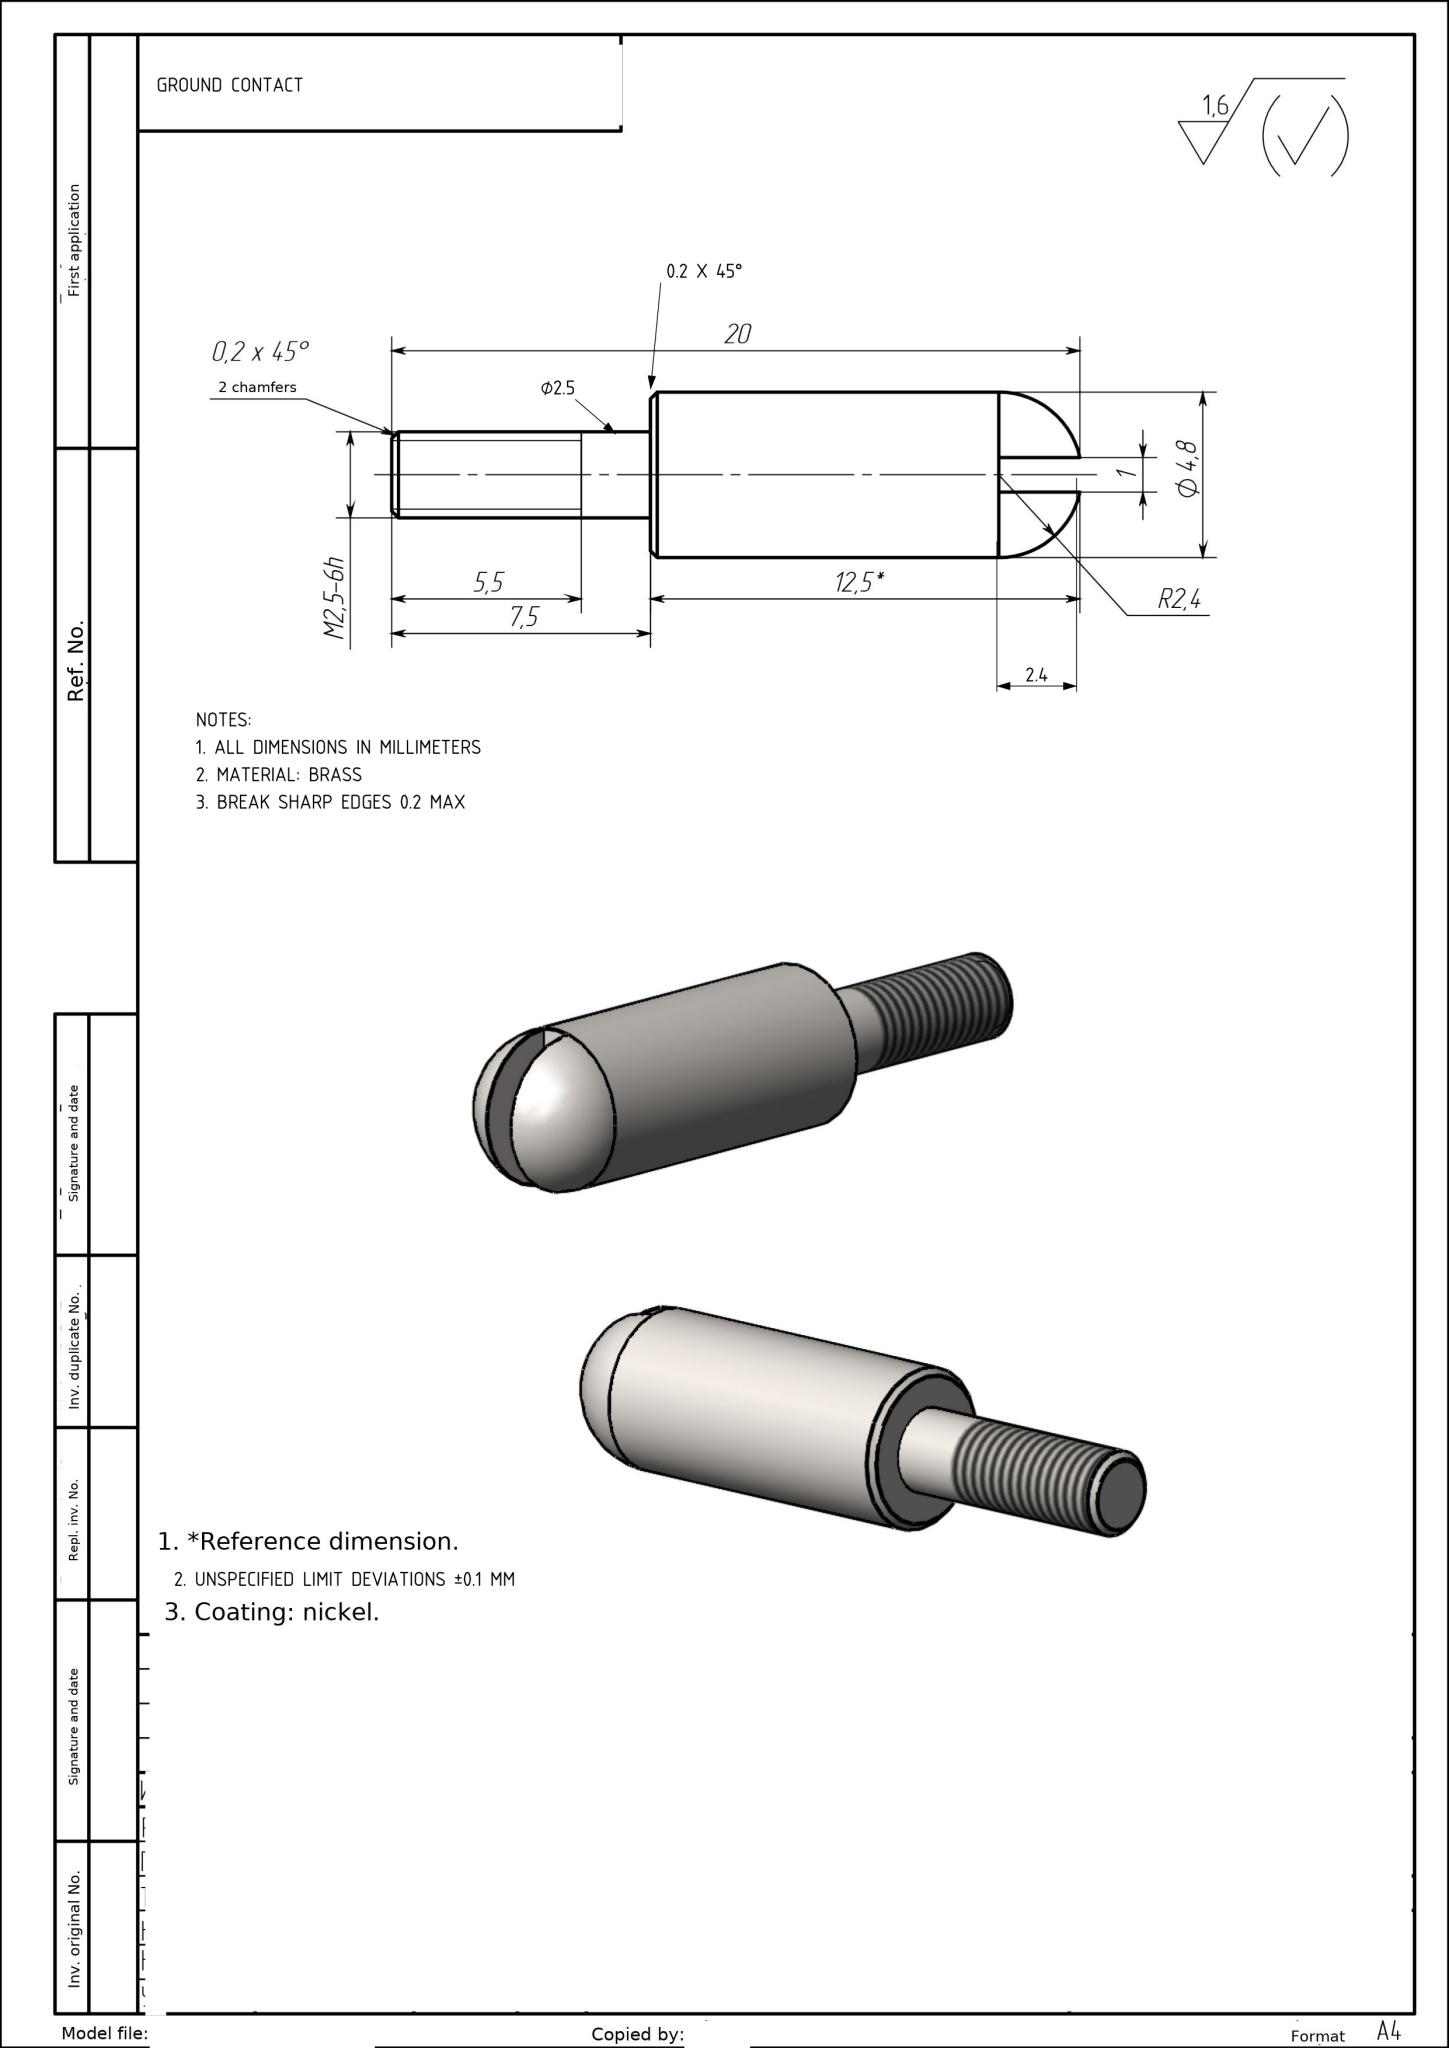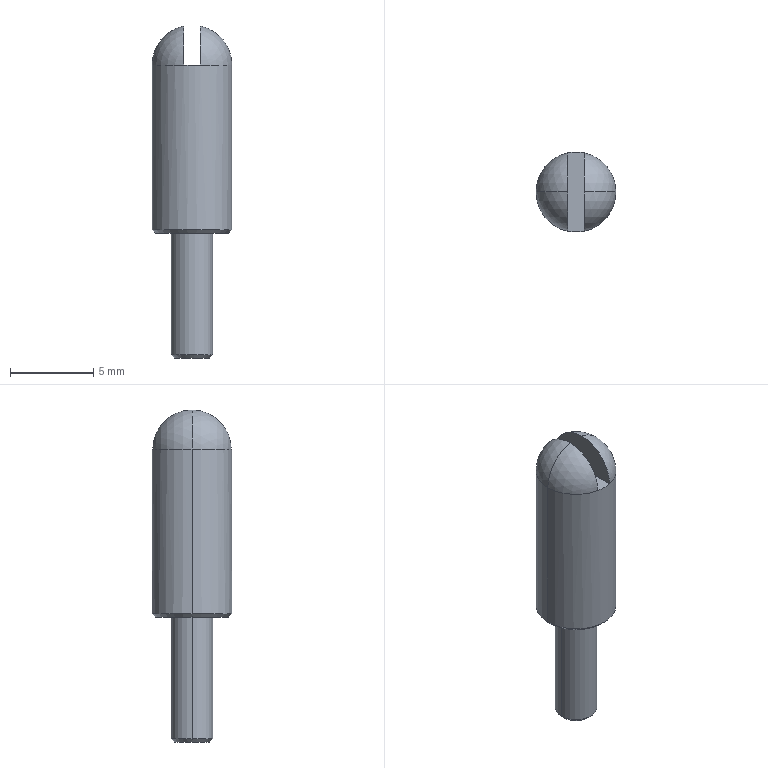Part | NX | mm | 1 solid | 17 faces | box 4.8 x 4.8 x 19.95 mm | volume 239 mm3 | plane 5 | cone 4 | sphere 4 | cylinder 4 | commonest cylinder face diameters 4.8 x2 2.5 x2
STEP:
#1=CARTESIAN_POINT('',(-2.2,0.,-12.5));
#2=VERTEX_POINT('',#1);
#3=CARTESIAN_POINT('',(2.2,0.,-12.5));
#4=VERTEX_POINT('',#3);
#5=CARTESIAN_POINT('',(0.,0.,-12.5));
#6=DIRECTION('',(0.,0.,-1.));
#7=DIRECTION('',(-1.,0.,0.));
#8=AXIS2_PLACEMENT_3D('',#5,#6,#7);
#9=CIRCLE('',#8,2.2);
#10=EDGE_CURVE('',#2,#4,#9,.T.);
#11=ORIENTED_EDGE('',*,*,#10,.F.);
#12=CARTESIAN_POINT('',(-2.4,0.,-12.3));
#13=VERTEX_POINT('',#12);
#14=CARTESIAN_POINT('',(-2.4,0.,-12.3));
#15=DIRECTION('',(-0.7071,0.,0.7071));
#16=VECTOR('',#15,1000.);
#17=LINE('',#14,#16);
#18=EDGE_CURVE('',#2,#13,#17,.T.);
#19=ORIENTED_EDGE('',*,*,#18,.T.);
#20=CARTESIAN_POINT('',(2.4,0.,-12.3));
#21=VERTEX_POINT('',#20);
#22=CARTESIAN_POINT('',(0.,0.,-12.3));
#23=DIRECTION('',(-0.,0.,1.));
#24=DIRECTION('',(-1.,0.,0.));
#25=AXIS2_PLACEMENT_3D('',#22,#23,#24);
#26=CIRCLE('',#25,2.4);
#27=EDGE_CURVE('',#21,#13,#26,.T.);
#28=ORIENTED_EDGE('',*,*,#27,.F.);
#29=CARTESIAN_POINT('',(2.4,0.,-12.3));
#30=DIRECTION('',(0.7071,0.,0.7071));
#31=VECTOR('',#30,1000.);
#32=LINE('',#29,#31);
#33=EDGE_CURVE('',#4,#21,#32,.T.);
#34=ORIENTED_EDGE('',*,*,#33,.F.);
#35=EDGE_LOOP('',(#11,#19,#28,#34));
#36=FACE_OUTER_BOUND('',#35,.T.);
#37=CARTESIAN_POINT('',(0.,0.,-12.3));
#38=DIRECTION('',(-0.,0.,1.));
#39=DIRECTION('',(1.,0.,0.));
#40=AXIS2_PLACEMENT_3D('',#37,#38,#39);
#41=CONICAL_SURFACE('',#40,2.4,0.7854);
#42=ADVANCED_FACE('',(#36),#41,.T.);
#43=CARTESIAN_POINT('',(-1.05,0.,-20.));
#44=VERTEX_POINT('',#43);
#45=CARTESIAN_POINT('',(1.05,0.,-20.));
#46=VERTEX_POINT('',#45);
#47=CARTESIAN_POINT('',(0.,0.,-20.));
#48=DIRECTION('',(0.,0.,-1.));
#49=DIRECTION('',(-1.,0.,0.));
#50=AXIS2_PLACEMENT_3D('',#47,#48,#49);
#51=CIRCLE('',#50,1.05);
#52=EDGE_CURVE('',#44,#46,#51,.T.);
#53=ORIENTED_EDGE('',*,*,#52,.F.);
#54=CARTESIAN_POINT('',(-1.25,0.,-19.8));
#55=VERTEX_POINT('',#54);
#56=CARTESIAN_POINT('',(-1.25,0.,-19.8));
#57=DIRECTION('',(-0.7071,0.,0.7071));
#58=VECTOR('',#57,1000.);
#59=LINE('',#56,#58);
#60=EDGE_CURVE('',#44,#55,#59,.T.);
#61=ORIENTED_EDGE('',*,*,#60,.T.);
#62=CARTESIAN_POINT('',(1.25,0.,-19.8));
#63=VERTEX_POINT('',#62);
#64=CARTESIAN_POINT('',(0.,0.,-19.8));
#65=DIRECTION('',(-0.,0.,1.));
#66=DIRECTION('',(-1.,0.,0.));
#67=AXIS2_PLACEMENT_3D('',#64,#65,#66);
#68=CIRCLE('',#67,1.25);
#69=EDGE_CURVE('',#63,#55,#68,.T.);
#70=ORIENTED_EDGE('',*,*,#69,.F.);
#71=CARTESIAN_POINT('',(1.25,0.,-19.8));
#72=DIRECTION('',(0.7071,0.,0.7071));
#73=VECTOR('',#72,1000.);
#74=LINE('',#71,#73);
#75=EDGE_CURVE('',#46,#63,#74,.T.);
#76=ORIENTED_EDGE('',*,*,#75,.F.);
#77=EDGE_LOOP('',(#53,#61,#70,#76));
#78=FACE_OUTER_BOUND('',#77,.T.);
#79=CARTESIAN_POINT('',(0.,0.,-19.8));
#80=DIRECTION('',(-0.,0.,1.));
#81=DIRECTION('',(1.,0.,0.));
#82=AXIS2_PLACEMENT_3D('',#79,#80,#81);
#83=CONICAL_SURFACE('',#82,1.25,0.7854);
#84=ADVANCED_FACE('',(#78),#83,.T.);
#85=CARTESIAN_POINT('',(2.4,0.,-2.4));
#86=VERTEX_POINT('',#85);
#87=CARTESIAN_POINT('',(0.5,-2.347,-2.4));
#88=VERTEX_POINT('',#87);
#89=CARTESIAN_POINT('',(0.,0.,-2.4));
#90=DIRECTION('',(0.,0.,-1.));
#91=DIRECTION('',(1.,0.,0.));
#92=AXIS2_PLACEMENT_3D('',#89,#90,#91);
#93=CIRCLE('',#92,2.4);
#94=EDGE_CURVE('',#86,#88,#93,.T.);
#95=ORIENTED_EDGE('',*,*,#94,.F.);
#96=CARTESIAN_POINT('',(0.5,0.,-0.05266));
#97=VERTEX_POINT('',#96);
#98=CARTESIAN_POINT('',(0.,0.,-2.4));
#99=DIRECTION('',(0.,-1.,0.));
#100=DIRECTION('',(0.,0.,-1.));
#101=AXIS2_PLACEMENT_3D('',#98,#99,#100);
#102=CIRCLE('',#101,2.4);
#103=EDGE_CURVE('',#86,#97,#102,.T.);
#104=ORIENTED_EDGE('',*,*,#103,.T.);
#105=CARTESIAN_POINT('',(0.5,-0.,-2.4));
#106=DIRECTION('',(-1.,0.,-0.));
#107=DIRECTION('',(0.,1.,0.));
#108=AXIS2_PLACEMENT_3D('',#105,#106,#107);
#109=CIRCLE('',#108,2.347);
#110=EDGE_CURVE('',#88,#97,#109,.T.);
#111=ORIENTED_EDGE('',*,*,#110,.F.);
#112=EDGE_LOOP('',(#95,#104,#111));
#113=FACE_OUTER_BOUND('',#112,.T.);
#114=CARTESIAN_POINT('',(0.,0.,-2.4));
#115=DIRECTION('',(0.,1.,0.));
#116=DIRECTION('',(1.,0.,0.));
#117=AXIS2_PLACEMENT_3D('',#114,#115,#116);
#118=SPHERICAL_SURFACE('',#117,2.4);
#119=ADVANCED_FACE('',(#113),#118,.T.);
#120=ORIENTED_EDGE('',*,*,#27,.T.);
#121=CARTESIAN_POINT('',(-2.4,0.,-2.4));
#122=VERTEX_POINT('',#121);
#123=CARTESIAN_POINT('',(-2.4,0.,-20.));
#124=DIRECTION('',(-0.,0.,1.));
#125=VECTOR('',#124,1000.);
#126=LINE('',#123,#125);
#127=EDGE_CURVE('',#13,#122,#126,.T.);
#128=ORIENTED_EDGE('',*,*,#127,.T.);
#129=CARTESIAN_POINT('',(-0.5,2.347,-2.4));
#130=VERTEX_POINT('',#129);
#131=CARTESIAN_POINT('',(0.,0.,-2.4));
#132=DIRECTION('',(0.,0.,-1.));
#133=DIRECTION('',(1.,0.,0.));
#134=AXIS2_PLACEMENT_3D('',#131,#132,#133);
#135=CIRCLE('',#134,2.4);
#136=EDGE_CURVE('',#122,#130,#135,.T.);
#137=ORIENTED_EDGE('',*,*,#136,.T.);
#138=CARTESIAN_POINT('',(0.5,2.347,-2.4));
#139=VERTEX_POINT('',#138);
#140=CARTESIAN_POINT('',(0.,0.,-2.4));
#141=DIRECTION('',(0.,0.,-1.));
#142=DIRECTION('',(1.,-0.,0.));
#143=AXIS2_PLACEMENT_3D('',#140,#141,#142);
#144=CIRCLE('',#143,2.4);
#145=EDGE_CURVE('',#130,#139,#144,.T.);
#146=ORIENTED_EDGE('',*,*,#145,.T.);
#147=CARTESIAN_POINT('',(0.,0.,-2.4));
#148=DIRECTION('',(0.,0.,-1.));
#149=DIRECTION('',(1.,0.,0.));
#150=AXIS2_PLACEMENT_3D('',#147,#148,#149);
#151=CIRCLE('',#150,2.4);
#152=EDGE_CURVE('',#139,#86,#151,.T.);
#153=ORIENTED_EDGE('',*,*,#152,.T.);
#154=CARTESIAN_POINT('',(2.4,0.,-20.));
#155=DIRECTION('',(-0.,0.,1.));
#156=VECTOR('',#155,1000.);
#157=LINE('',#154,#156);
#158=EDGE_CURVE('',#21,#86,#157,.T.);
#159=ORIENTED_EDGE('',*,*,#158,.F.);
#160=EDGE_LOOP('',(#120,#128,#137,#146,#153,#159));
#161=FACE_OUTER_BOUND('',#160,.T.);
#162=CARTESIAN_POINT('',(0.,0.,-20.));
#163=DIRECTION('',(-0.,0.,1.));
#164=DIRECTION('',(1.,0.,0.));
#165=AXIS2_PLACEMENT_3D('',#162,#163,#164);
#166=CYLINDRICAL_SURFACE('',#165,2.4);
#167=ADVANCED_FACE('',(#161),#166,.T.);
#168=ORIENTED_EDGE('',*,*,#69,.T.);
#169=CARTESIAN_POINT('',(-1.25,0.,-12.5));
#170=VERTEX_POINT('',#169);
#171=CARTESIAN_POINT('',(-1.25,0.,-20.));
#172=DIRECTION('',(-0.,0.,1.));
#173=VECTOR('',#172,1000.);
#174=LINE('',#171,#173);
#175=EDGE_CURVE('',#55,#170,#174,.T.);
#176=ORIENTED_EDGE('',*,*,#175,.T.);
#177=CARTESIAN_POINT('',(1.25,0.,-12.5));
#178=VERTEX_POINT('',#177);
#179=CARTESIAN_POINT('',(0.,0.,-12.5));
#180=DIRECTION('',(-0.,0.,1.));
#181=DIRECTION('',(1.,0.,0.));
#182=AXIS2_PLACEMENT_3D('',#179,#180,#181);
#183=CIRCLE('',#182,1.25);
#184=EDGE_CURVE('',#178,#170,#183,.T.);
#185=ORIENTED_EDGE('',*,*,#184,.F.);
#186=CARTESIAN_POINT('',(1.25,0.,-20.));
#187=DIRECTION('',(-0.,0.,1.));
#188=VECTOR('',#187,1000.);
#189=LINE('',#186,#188);
#190=EDGE_CURVE('',#63,#178,#189,.T.);
#191=ORIENTED_EDGE('',*,*,#190,.F.);
#192=EDGE_LOOP('',(#168,#176,#185,#191));
#193=FACE_OUTER_BOUND('',#192,.T.);
#194=CARTESIAN_POINT('',(0.,0.,-20.));
#195=DIRECTION('',(-0.,0.,1.));
#196=DIRECTION('',(1.,0.,0.));
#197=AXIS2_PLACEMENT_3D('',#194,#195,#196);
#198=CYLINDRICAL_SURFACE('',#197,1.25);
#199=ADVANCED_FACE('',(#193),#198,.T.);
#200=ORIENTED_EDGE('',*,*,#136,.F.);
#201=CARTESIAN_POINT('',(-0.5,0.,-0.05266));
#202=VERTEX_POINT('',#201);
#203=CARTESIAN_POINT('',(0.,0.,-2.4));
#204=DIRECTION('',(0.,1.,0.));
#205=DIRECTION('',(-1.,0.,0.));
#206=AXIS2_PLACEMENT_3D('',#203,#204,#205);
#207=CIRCLE('',#206,2.4);
#208=EDGE_CURVE('',#122,#202,#207,.T.);
#209=ORIENTED_EDGE('',*,*,#208,.T.);
#210=CARTESIAN_POINT('',(-0.5,0.,-2.4));
#211=DIRECTION('',(1.,0.,0.));
#212=DIRECTION('',(-0.,0.,1.));
#213=AXIS2_PLACEMENT_3D('',#210,#211,#212);
#214=CIRCLE('',#213,2.347);
#215=EDGE_CURVE('',#130,#202,#214,.T.);
#216=ORIENTED_EDGE('',*,*,#215,.F.);
#217=EDGE_LOOP('',(#200,#209,#216));
#218=FACE_OUTER_BOUND('',#217,.T.);
#219=CARTESIAN_POINT('',(0.,0.,-2.4));
#220=DIRECTION('',(0.,1.,0.));
#221=DIRECTION('',(1.,0.,0.));
#222=AXIS2_PLACEMENT_3D('',#219,#220,#221);
#223=SPHERICAL_SURFACE('',#222,2.4);
#224=ADVANCED_FACE('',(#218),#223,.T.);
#225=ORIENTED_EDGE('',*,*,#208,.F.);
#226=CARTESIAN_POINT('',(-0.5,-2.347,-2.4));
#227=VERTEX_POINT('',#226);
#228=CARTESIAN_POINT('',(0.,0.,-2.4));
#229=DIRECTION('',(0.,0.,-1.));
#230=DIRECTION('',(1.,0.,0.));
#231=AXIS2_PLACEMENT_3D('',#228,#229,#230);
#232=CIRCLE('',#231,2.4);
#233=EDGE_CURVE('',#227,#122,#232,.T.);
#234=ORIENTED_EDGE('',*,*,#233,.F.);
#235=CARTESIAN_POINT('',(-0.5,0.,-2.4));
#236=DIRECTION('',(1.,0.,0.));
#237=DIRECTION('',(-0.,0.,1.));
#238=AXIS2_PLACEMENT_3D('',#235,#236,#237);
#239=CIRCLE('',#238,2.347);
#240=EDGE_CURVE('',#202,#227,#239,.T.);
#241=ORIENTED_EDGE('',*,*,#240,.F.);
#242=EDGE_LOOP('',(#225,#234,#241));
#243=FACE_OUTER_BOUND('',#242,.T.);
#244=CARTESIAN_POINT('',(0.,0.,-2.4));
#245=DIRECTION('',(0.,1.,0.));
#246=DIRECTION('',(1.,0.,0.));
#247=AXIS2_PLACEMENT_3D('',#244,#245,#246);
#248=SPHERICAL_SURFACE('',#247,2.4);
#249=ADVANCED_FACE('',(#243),#248,.T.);
#250=ORIENTED_EDGE('',*,*,#175,.F.);
#251=CARTESIAN_POINT('',(0.,0.,-19.8));
#252=DIRECTION('',(-0.,0.,1.));
#253=DIRECTION('',(-1.,0.,0.));
#254=AXIS2_PLACEMENT_3D('',#251,#252,#253);
#255=CIRCLE('',#254,1.25);
#256=EDGE_CURVE('',#55,#63,#255,.T.);
#257=ORIENTED_EDGE('',*,*,#256,.T.);
#258=ORIENTED_EDGE('',*,*,#190,.T.);
#259=CARTESIAN_POINT('',(0.,0.,-12.5));
#260=DIRECTION('',(-0.,0.,1.));
#261=DIRECTION('',(1.,0.,0.));
#262=AXIS2_PLACEMENT_3D('',#259,#260,#261);
#263=CIRCLE('',#262,1.25);
#264=EDGE_CURVE('',#170,#178,#263,.T.);
#265=ORIENTED_EDGE('',*,*,#264,.F.);
#266=EDGE_LOOP('',(#250,#257,#258,#265));
#267=FACE_OUTER_BOUND('',#266,.T.);
#268=CARTESIAN_POINT('',(0.,0.,-20.));
#269=DIRECTION('',(-0.,0.,1.));
#270=DIRECTION('',(1.,0.,0.));
#271=AXIS2_PLACEMENT_3D('',#268,#269,#270);
#272=CYLINDRICAL_SURFACE('',#271,1.25);
#273=ADVANCED_FACE('',(#267),#272,.T.);
#274=CARTESIAN_POINT('',(0.,0.,-20.));
#275=DIRECTION('',(0.,0.,-1.));
#276=DIRECTION('',(-1.,0.,0.));
#277=AXIS2_PLACEMENT_3D('',#274,#275,#276);
#278=CIRCLE('',#277,1.05);
#279=EDGE_CURVE('',#46,#44,#278,.T.);
#280=ORIENTED_EDGE('',*,*,#279,.T.);
#281=ORIENTED_EDGE('',*,*,#52,.T.);
#282=EDGE_LOOP('',(#280,#281));
#283=FACE_OUTER_BOUND('',#282,.T.);
#284=CARTESIAN_POINT('',(1.25,0.,-20.));
#285=DIRECTION('',(0.,0.,-1.));
#286=DIRECTION('',(-1.,0.,-0.));
#287=AXIS2_PLACEMENT_3D('',#284,#285,#286);
#288=PLANE('',#287);
#289=ADVANCED_FACE('',(#283),#288,.T.);
#290=ORIENTED_EDGE('',*,*,#127,.F.);
#291=CARTESIAN_POINT('',(0.,0.,-12.3));
#292=DIRECTION('',(-0.,0.,1.));
#293=DIRECTION('',(-1.,0.,0.));
#294=AXIS2_PLACEMENT_3D('',#291,#292,#293);
#295=CIRCLE('',#294,2.4);
#296=EDGE_CURVE('',#13,#21,#295,.T.);
#297=ORIENTED_EDGE('',*,*,#296,.T.);
#298=ORIENTED_EDGE('',*,*,#158,.T.);
#299=ORIENTED_EDGE('',*,*,#94,.T.);
#300=CARTESIAN_POINT('',(0.,0.,-2.4));
#301=DIRECTION('',(0.,0.,-1.));
#302=DIRECTION('',(1.,0.,0.));
#303=AXIS2_PLACEMENT_3D('',#300,#301,#302);
#304=CIRCLE('',#303,2.4);
#305=EDGE_CURVE('',#88,#227,#304,.T.);
#306=ORIENTED_EDGE('',*,*,#305,.T.);
#307=ORIENTED_EDGE('',*,*,#233,.T.);
#308=EDGE_LOOP('',(#290,#297,#298,#299,#306,#307));
#309=FACE_OUTER_BOUND('',#308,.T.);
#310=CARTESIAN_POINT('',(0.,0.,-20.));
#311=DIRECTION('',(-0.,0.,1.));
#312=DIRECTION('',(1.,0.,0.));
#313=AXIS2_PLACEMENT_3D('',#310,#311,#312);
#314=CYLINDRICAL_SURFACE('',#313,2.4);
#315=ADVANCED_FACE('',(#309),#314,.T.);
#316=CARTESIAN_POINT('',(0.,0.,-12.5));
#317=DIRECTION('',(0.,0.,-1.));
#318=DIRECTION('',(-1.,0.,0.));
#319=AXIS2_PLACEMENT_3D('',#316,#317,#318);
#320=CIRCLE('',#319,2.2);
#321=EDGE_CURVE('',#4,#2,#320,.T.);
#322=ORIENTED_EDGE('',*,*,#321,.T.);
#323=ORIENTED_EDGE('',*,*,#10,.T.);
#324=EDGE_LOOP('',(#322,#323));
#325=FACE_OUTER_BOUND('',#324,.T.);
#326=ORIENTED_EDGE('',*,*,#184,.T.);
#327=ORIENTED_EDGE('',*,*,#264,.T.);
#328=EDGE_LOOP('',(#326,#327));
#329=FACE_BOUND('',#328,.T.);
#330=CARTESIAN_POINT('',(2.4,0.,-12.5));
#331=DIRECTION('',(0.,0.,-1.));
#332=DIRECTION('',(-1.,0.,-0.));
#333=AXIS2_PLACEMENT_3D('',#330,#331,#332);
#334=PLANE('',#333);
#335=ADVANCED_FACE('',(#325,#329),#334,.T.);
#336=ORIENTED_EDGE('',*,*,#103,.F.);
#337=ORIENTED_EDGE('',*,*,#152,.F.);
#338=CARTESIAN_POINT('',(0.5,-0.,-2.4));
#339=DIRECTION('',(-1.,0.,-0.));
#340=DIRECTION('',(0.,1.,0.));
#341=AXIS2_PLACEMENT_3D('',#338,#339,#340);
#342=CIRCLE('',#341,2.347);
#343=EDGE_CURVE('',#97,#139,#342,.T.);
#344=ORIENTED_EDGE('',*,*,#343,.F.);
#345=EDGE_LOOP('',(#336,#337,#344));
#346=FACE_OUTER_BOUND('',#345,.T.);
#347=CARTESIAN_POINT('',(0.,0.,-2.4));
#348=DIRECTION('',(0.,1.,0.));
#349=DIRECTION('',(1.,0.,0.));
#350=AXIS2_PLACEMENT_3D('',#347,#348,#349);
#351=SPHERICAL_SURFACE('',#350,2.4);
#352=ADVANCED_FACE('',(#346),#351,.T.);
#353=ORIENTED_EDGE('',*,*,#60,.F.);
#354=ORIENTED_EDGE('',*,*,#279,.F.);
#355=ORIENTED_EDGE('',*,*,#75,.T.);
#356=ORIENTED_EDGE('',*,*,#256,.F.);
#357=EDGE_LOOP('',(#353,#354,#355,#356));
#358=FACE_OUTER_BOUND('',#357,.T.);
#359=CARTESIAN_POINT('',(0.,0.,-19.8));
#360=DIRECTION('',(-0.,0.,1.));
#361=DIRECTION('',(1.,0.,0.));
#362=AXIS2_PLACEMENT_3D('',#359,#360,#361);
#363=CONICAL_SURFACE('',#362,1.25,0.7854);
#364=ADVANCED_FACE('',(#358),#363,.T.);
#365=ORIENTED_EDGE('',*,*,#18,.F.);
#366=ORIENTED_EDGE('',*,*,#321,.F.);
#367=ORIENTED_EDGE('',*,*,#33,.T.);
#368=ORIENTED_EDGE('',*,*,#296,.F.);
#369=EDGE_LOOP('',(#365,#366,#367,#368));
#370=FACE_OUTER_BOUND('',#369,.T.);
#371=CARTESIAN_POINT('',(0.,0.,-12.3));
#372=DIRECTION('',(-0.,0.,1.));
#373=DIRECTION('',(1.,0.,0.));
#374=AXIS2_PLACEMENT_3D('',#371,#372,#373);
#375=CONICAL_SURFACE('',#374,2.4,0.7854);
#376=ADVANCED_FACE('',(#370),#375,.T.);
#377=ORIENTED_EDGE('',*,*,#215,.T.);
#378=ORIENTED_EDGE('',*,*,#240,.T.);
#379=CARTESIAN_POINT('',(-0.5,-2.4,-2.4));
#380=DIRECTION('',(0.,1.,0.));
#381=VECTOR('',#380,1000.);
#382=LINE('',#379,#381);
#383=EDGE_CURVE('',#227,#130,#382,.T.);
#384=ORIENTED_EDGE('',*,*,#383,.T.);
#385=EDGE_LOOP('',(#377,#378,#384));
#386=FACE_OUTER_BOUND('',#385,.T.);
#387=CARTESIAN_POINT('',(-0.5,-2.4,7.6));
#388=DIRECTION('',(-1.,0.,-0.));
#389=DIRECTION('',(-0.,0.,1.));
#390=AXIS2_PLACEMENT_3D('',#387,#388,#389);
#391=PLANE('',#390);
#392=ADVANCED_FACE('',(#386),#391,.F.);
#393=ORIENTED_EDGE('',*,*,#110,.T.);
#394=ORIENTED_EDGE('',*,*,#343,.T.);
#395=CARTESIAN_POINT('',(0.5,-2.4,-2.4));
#396=DIRECTION('',(-0.,-1.,0.));
#397=VECTOR('',#396,1000.);
#398=LINE('',#395,#397);
#399=EDGE_CURVE('',#139,#88,#398,.T.);
#400=ORIENTED_EDGE('',*,*,#399,.T.);
#401=EDGE_LOOP('',(#393,#394,#400));
#402=FACE_OUTER_BOUND('',#401,.T.);
#403=CARTESIAN_POINT('',(0.5,-2.4,7.6));
#404=DIRECTION('',(1.,-0.,0.));
#405=DIRECTION('',(0.,1.,0.));
#406=AXIS2_PLACEMENT_3D('',#403,#404,#405);
#407=PLANE('',#406);
#408=ADVANCED_FACE('',(#402),#407,.F.);
#409=ORIENTED_EDGE('',*,*,#399,.F.);
#410=ORIENTED_EDGE('',*,*,#145,.F.);
#411=ORIENTED_EDGE('',*,*,#383,.F.);
#412=ORIENTED_EDGE('',*,*,#305,.F.);
#413=EDGE_LOOP('',(#409,#410,#411,#412));
#414=FACE_OUTER_BOUND('',#413,.T.);
#415=CARTESIAN_POINT('',(-0.,0.,-2.4));
#416=DIRECTION('',(0.,0.,1.));
#417=DIRECTION('',(1.,0.,0.));
#418=AXIS2_PLACEMENT_3D('',#415,#416,#417);
#419=PLANE('',#418);
#420=ADVANCED_FACE('',(#414),#419,.T.);
#421=CLOSED_SHELL('',(#42,#84,#119,#167,#199,#224,#249,#273,#289,#315,#335,#352,#364,#376,#392,#408,#420));
#422=MANIFOLD_SOLID_BREP('',#421);
#423=CARTESIAN_POINT('',(0.,0.,0.));
#424=DIRECTION('',(0.,0.,1.));
#425=DIRECTION('',(1.,0.,0.));
#426=AXIS2_PLACEMENT_3D('',#423,#424,#425);
#427=(LENGTH_UNIT()NAMED_UNIT(*)SI_UNIT(.MILLI.,.METRE.));
#428=UNCERTAINTY_MEASURE_WITH_UNIT(LENGTH_MEASURE(0.00001),#427,'','');
#429=(NAMED_UNIT(*)PLANE_ANGLE_UNIT()SI_UNIT($,.RADIAN.));
#430=(NAMED_UNIT(*)SI_UNIT($,.STERADIAN.)SOLID_ANGLE_UNIT());
#431=(GEOMETRIC_REPRESENTATION_CONTEXT(3)GLOBAL_UNCERTAINTY_ASSIGNED_CONTEXT((#428))GLOBAL_UNIT_ASSIGNED_CONTEXT((#427,#429,#430))REPRESENTATION_CONTEXT('',''));
#432=ADVANCED_BREP_SHAPE_REPRESENTATION('',(#422,#426),#431);